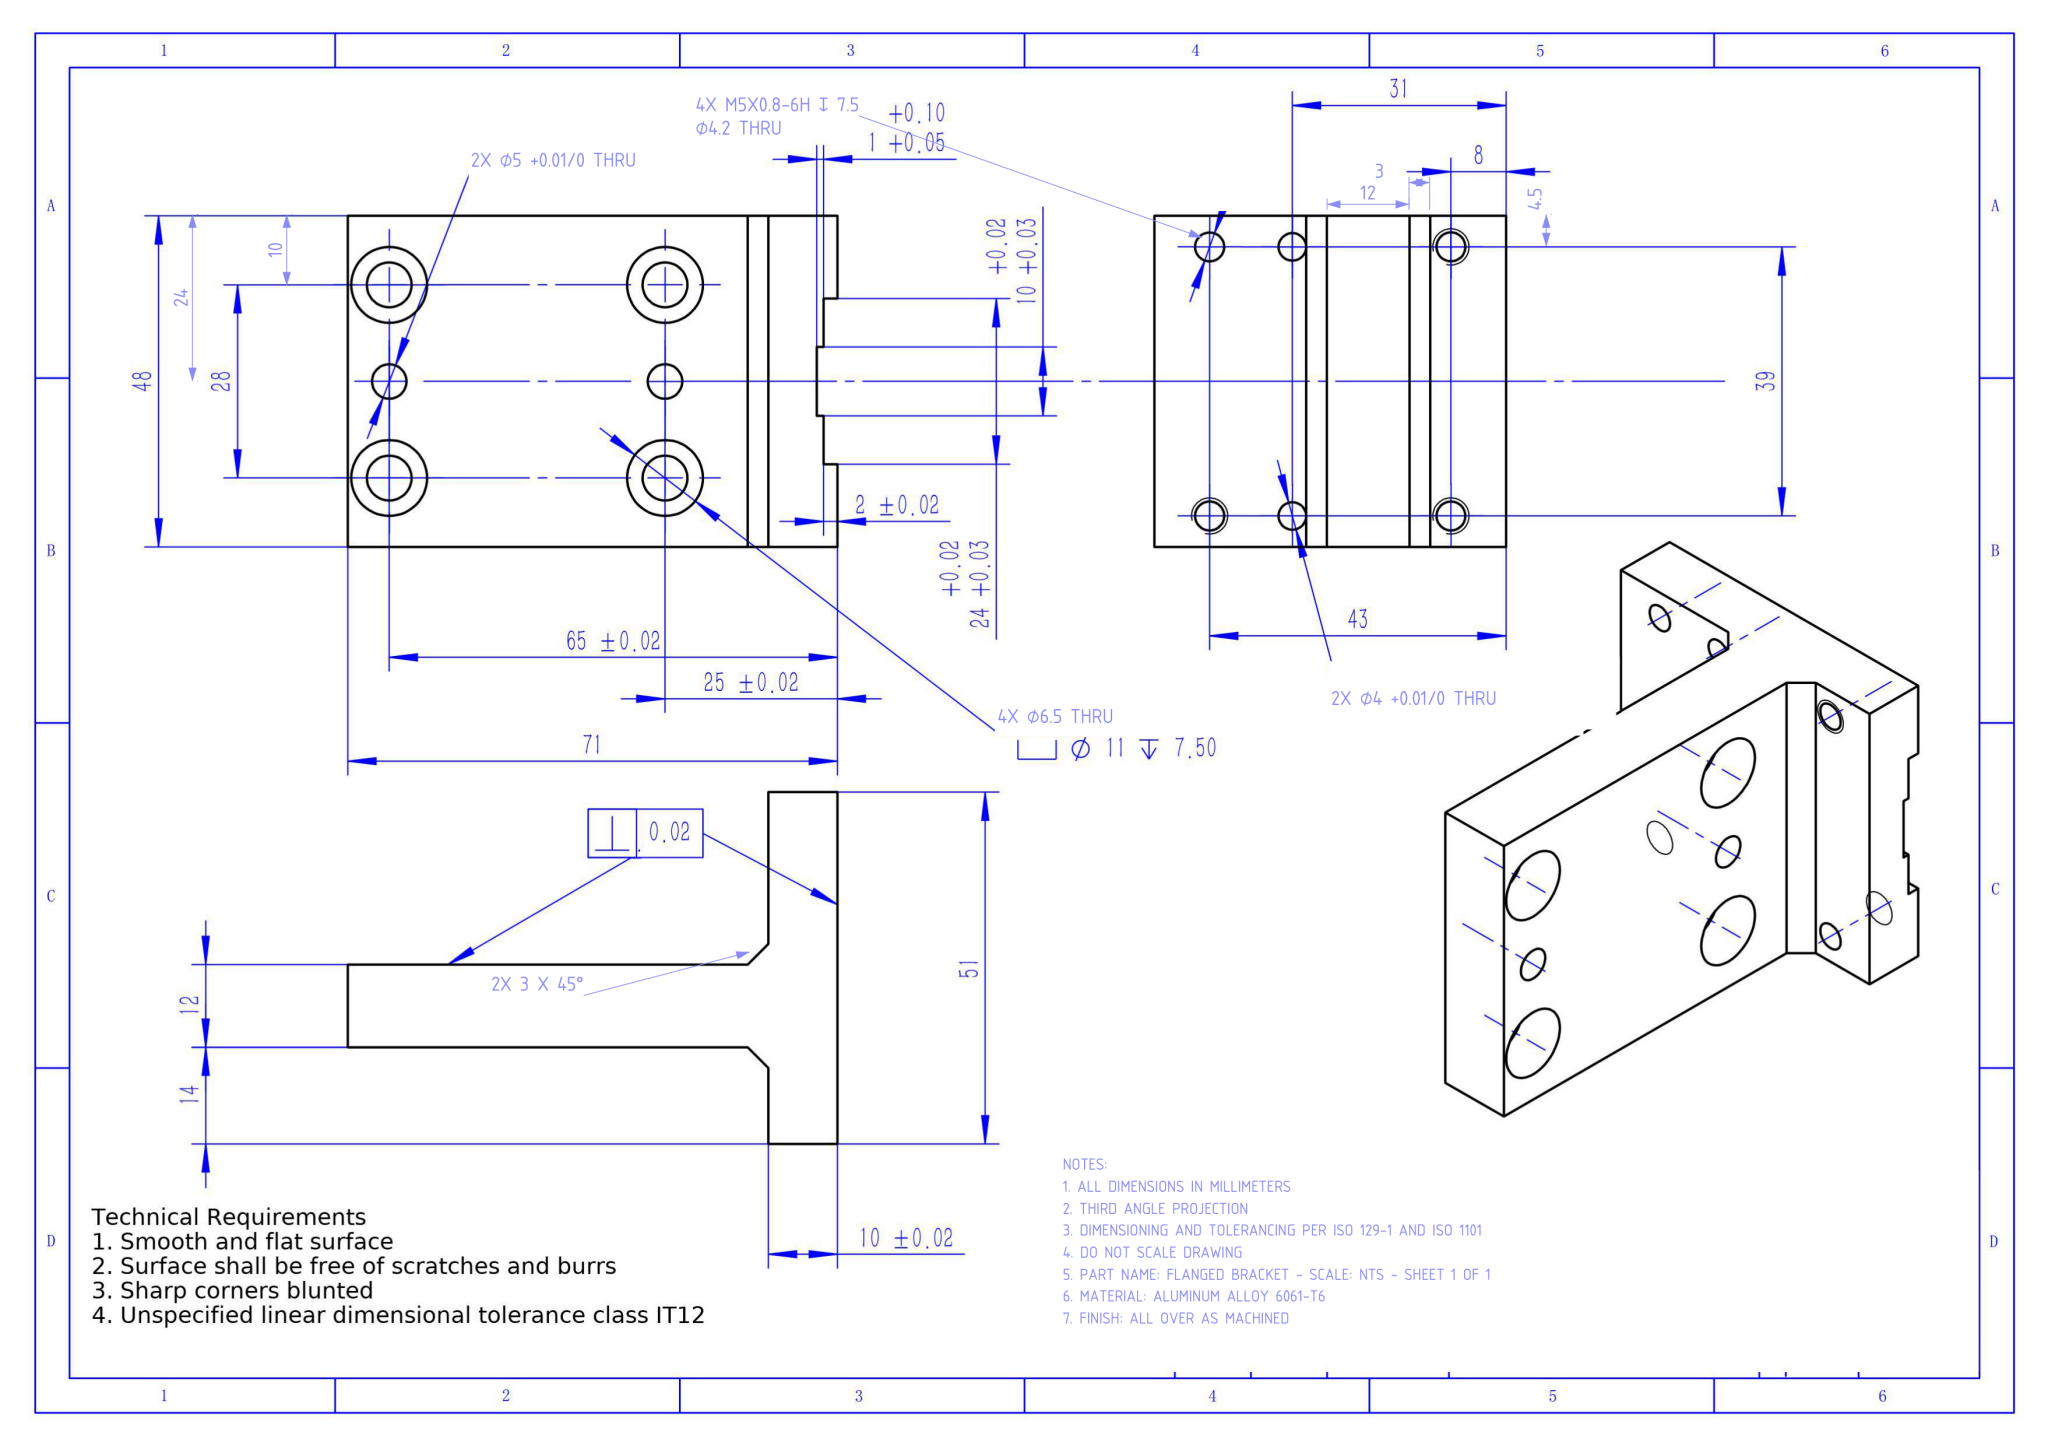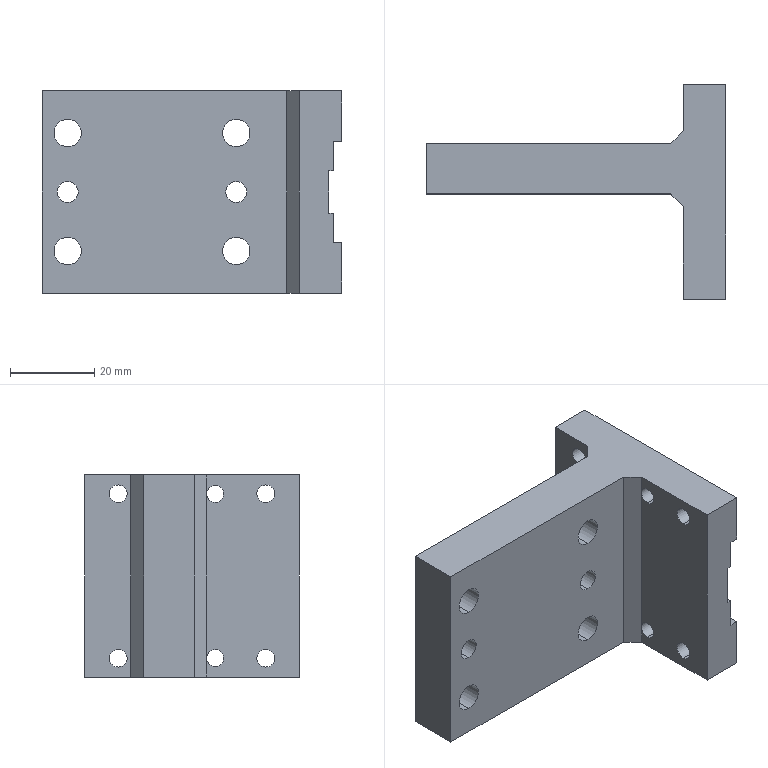Part | NX | mm | 1 solid | 56 faces | box 71 x 51 x 48 mm | volume 52365 mm3 | cylinder 32 | plane 24 | commonest cylinder face diameters 4.2 x8 11 x8 6.5 x8 4 x4 5 x4